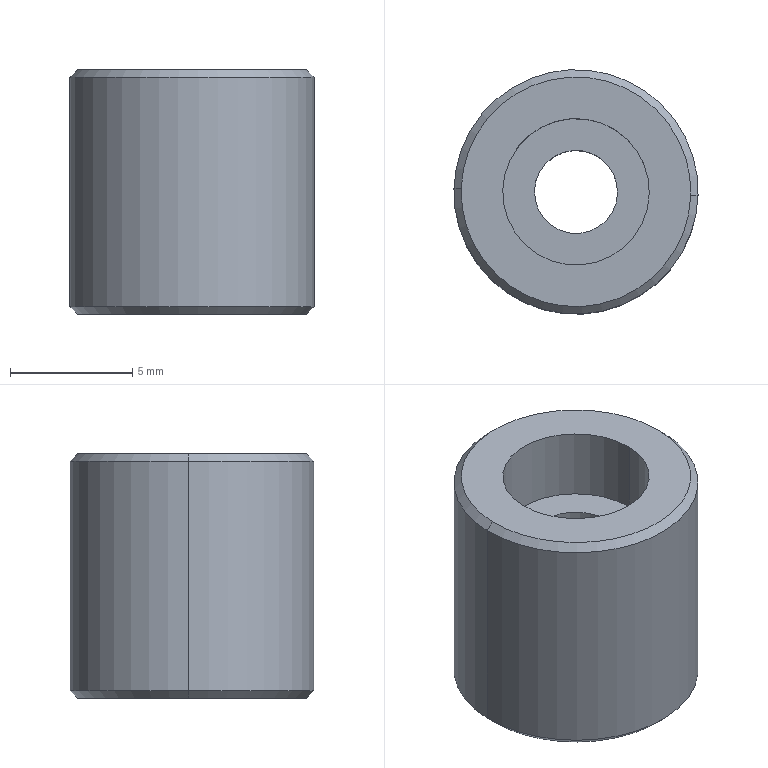Component | SolidWorks | DZ.KX.203-TC1505-20-18-05-90-1 | 1 solid | 15 faces | box 10 x 10 x 10 mm | volume 623 mm3 | cone 6 | cylinder 6 | plane 3 | commonest cylinder face diameters 3.4 x2 6 x2 10 x2 | material Plain Carbon Steel
build123d program:
from build123d import *

# Parameters (mm, degrees)
SKETCH1_R                                            = 5
BOSS_EXTRUDE1_DEPTH                                  = 10
F_6_0_6_DIAMETER_HOLE1_D                             = 6
F_6_0_6_DIAMETER_HOLE1_DEPTH                         = 3
HOLE_SIZE_SLOTTED_RAISED_COUNTERSUNK_SCR_D           = 3.4
HOLE_SIZE_SLOTTED_RAISED_COUNTERSUNK_SCR_CSINK_D     = 6
HOLE_SIZE_SLOTTED_RAISED_COUNTERSUNK_SCR_CSINK_ANGLE = 90
CHAMFER1_SIZE                                        = 0.3


with BuildPart() as part:
    # Sketch1 → Boss-Extrude1 (new body)
    with BuildSketch(Plane(origin=(0, 0, 0), x_dir=(0, 0, -1), z_dir=(1, 0, 0))):
        Circle(SKETCH1_R)
    extrude(amount=BOSS_EXTRUDE1_DEPTH)

    # 6.0 _6_ Diameter Hole1
    with Locations(Plane(origin=(10, 0, 0), x_dir=(0, 0, -1), z_dir=(1, 0, 0))):
        with Locations((0, 0)):
            Hole(F_6_0_6_DIAMETER_HOLE1_D / 2, depth=F_6_0_6_DIAMETER_HOLE1_DEPTH)

    # Hole Size Slotted Raised Countersunk Scr (through all)
    with Locations(Plane.ZY):
        with Locations((0, 0)):
            CounterSinkHole(HOLE_SIZE_SLOTTED_RAISED_COUNTERSUNK_SCR_D / 2, HOLE_SIZE_SLOTTED_RAISED_COUNTERSUNK_SCR_CSINK_D / 2, counter_sink_angle=HOLE_SIZE_SLOTTED_RAISED_COUNTERSUNK_SCR_CSINK_ANGLE)

    # Chamfer1
    chamfer1_edges = [part.edges().sort_by_distance(p)[0] for p in [
        (0, 0, 5),
        (10, 0, 5),
    ]]
    chamfer(chamfer1_edges, length=CHAMFER1_SIZE)


solid = part.part

# Placed as in the assembly
solid = solid.moved(Location((295.5, -817.807, 17.06), (0, -90, 0)))
STEP:
#1=COLOUR_RGB('',0.7922,0.8196,0.9333);
#2=FILL_AREA_STYLE_COLOUR('',#1);
#3=FILL_AREA_STYLE('',(#2));
#4=SURFACE_STYLE_FILL_AREA(#3);
#5=SURFACE_SIDE_STYLE('',(#4));
#6=SURFACE_STYLE_USAGE(.BOTH.,#5);
#7=PRESENTATION_STYLE_ASSIGNMENT((#6));
#8=CARTESIAN_POINT('',(11.819,-32.203,1.065));
#9=VERTEX_POINT('',#8);
#10=CARTESIAN_POINT('',(11.449,-32.192,1.065));
#11=VERTEX_POINT('',#10);
#12=CARTESIAN_POINT('',(11.634,-32.197,1.065));
#13=DIRECTION('',(0.,0.,1.));
#14=DIRECTION('',(0.9996,-0.02934,0.));
#15=AXIS2_PLACEMENT_3D('',#12,#13,#14);
#16=CIRCLE('',#15,0.185);
#17=EDGE_CURVE('',#9,#11,#16,.T.);
#18=ORIENTED_EDGE('',*,*,#17,.F.);
#19=CARTESIAN_POINT('',(11.831,-32.203,1.054));
#20=VERTEX_POINT('',#19);
#21=CARTESIAN_POINT('',(11.819,-32.203,1.065));
#22=DIRECTION('',(0.7068,-0.02075,-0.7071));
#23=VECTOR('',#22,39.37);
#24=LINE('',#21,#23);
#25=EDGE_CURVE('',#9,#20,#24,.T.);
#26=ORIENTED_EDGE('',*,*,#25,.T.);
#27=CARTESIAN_POINT('',(11.437,-32.191,1.054));
#28=VERTEX_POINT('',#27);
#29=CARTESIAN_POINT('',(11.634,-32.197,1.054));
#30=DIRECTION('',(-0.,-0.,-1.));
#31=DIRECTION('',(0.9996,-0.02934,0.));
#32=AXIS2_PLACEMENT_3D('',#29,#30,#31);
#33=CIRCLE('',#32,0.1969);
#34=EDGE_CURVE('',#28,#20,#33,.T.);
#35=ORIENTED_EDGE('',*,*,#34,.F.);
#36=CARTESIAN_POINT('',(11.449,-32.192,1.065));
#37=DIRECTION('',(-0.7068,0.02075,-0.7071));
#38=VECTOR('',#37,39.37);
#39=LINE('',#36,#38);
#40=EDGE_CURVE('',#11,#28,#39,.T.);
#41=ORIENTED_EDGE('',*,*,#40,.F.);
#42=EDGE_LOOP('',(#18,#26,#35,#41));
#43=FACE_OUTER_BOUND('',#42,.T.);
#44=CARTESIAN_POINT('',(11.634,-32.197,1.065));
#45=DIRECTION('',(-0.,-0.,-1.));
#46=DIRECTION('',(-0.9996,0.02934,0.));
#47=AXIS2_PLACEMENT_3D('',#44,#45,#46);
#48=CONICAL_SURFACE('',#47,0.185,0.7854);
#49=ADVANCED_FACE('',(#43),#48,.T.);
#50=CARTESIAN_POINT('',(11.449,-32.192,0.6716));
#51=VERTEX_POINT('',#50);
#52=CARTESIAN_POINT('',(11.819,-32.203,0.6716));
#53=VERTEX_POINT('',#52);
#54=CARTESIAN_POINT('',(11.634,-32.197,0.6716));
#55=DIRECTION('',(-0.,-0.,-1.));
#56=DIRECTION('',(0.9996,-0.02934,0.));
#57=AXIS2_PLACEMENT_3D('',#54,#55,#56);
#58=CIRCLE('',#57,0.185);
#59=EDGE_CURVE('',#51,#53,#58,.T.);
#60=ORIENTED_EDGE('',*,*,#59,.F.);
#61=CARTESIAN_POINT('',(11.437,-32.191,0.6834));
#62=VERTEX_POINT('',#61);
#63=CARTESIAN_POINT('',(11.437,-32.191,0.6834));
#64=DIRECTION('',(-0.7068,0.02075,0.7071));
#65=VECTOR('',#64,39.37);
#66=LINE('',#63,#65);
#67=EDGE_CURVE('',#51,#62,#66,.T.);
#68=ORIENTED_EDGE('',*,*,#67,.T.);
#69=CARTESIAN_POINT('',(11.831,-32.203,0.6834));
#70=VERTEX_POINT('',#69);
#71=CARTESIAN_POINT('',(11.634,-32.197,0.6834));
#72=DIRECTION('',(0.,0.,1.));
#73=DIRECTION('',(0.9996,-0.02934,0.));
#74=AXIS2_PLACEMENT_3D('',#71,#72,#73);
#75=CIRCLE('',#74,0.1969);
#76=EDGE_CURVE('',#70,#62,#75,.T.);
#77=ORIENTED_EDGE('',*,*,#76,.F.);
#78=CARTESIAN_POINT('',(11.831,-32.203,0.6834));
#79=DIRECTION('',(0.7068,-0.02075,0.7071));
#80=VECTOR('',#79,39.37);
#81=LINE('',#78,#80);
#82=EDGE_CURVE('',#53,#70,#81,.T.);
#83=ORIENTED_EDGE('',*,*,#82,.F.);
#84=EDGE_LOOP('',(#60,#68,#77,#83));
#85=FACE_OUTER_BOUND('',#84,.T.);
#86=CARTESIAN_POINT('',(11.634,-32.197,0.6834));
#87=DIRECTION('',(0.,0.,1.));
#88=DIRECTION('',(0.9996,-0.02934,0.));
#89=AXIS2_PLACEMENT_3D('',#86,#87,#88);
#90=CONICAL_SURFACE('',#89,0.1969,0.7854);
#91=ADVANCED_FACE('',(#85),#90,.T.);
#92=CARTESIAN_POINT('',(11.701,-32.199,0.7228));
#93=VERTEX_POINT('',#92);
#94=CARTESIAN_POINT('',(11.567,-32.195,0.7228));
#95=VERTEX_POINT('',#94);
#96=CARTESIAN_POINT('',(11.634,-32.197,0.7228));
#97=DIRECTION('',(-0.,-0.,-1.));
#98=DIRECTION('',(-0.9996,0.02934,0.));
#99=AXIS2_PLACEMENT_3D('',#96,#97,#98);
#100=CIRCLE('',#99,0.06693);
#101=EDGE_CURVE('',#93,#95,#100,.T.);
#102=ORIENTED_EDGE('',*,*,#101,.F.);
#103=CARTESIAN_POINT('',(11.752,-32.201,0.6716));
#104=VERTEX_POINT('',#103);
#105=CARTESIAN_POINT('',(11.752,-32.201,0.6716));
#106=DIRECTION('',(0.7068,-0.02075,-0.7071));
#107=VECTOR('',#106,39.37);
#108=LINE('',#105,#107);
#109=EDGE_CURVE('',#93,#104,#108,.T.);
#110=ORIENTED_EDGE('',*,*,#109,.T.);
#111=CARTESIAN_POINT('',(11.516,-32.194,0.6716));
#112=VERTEX_POINT('',#111);
#113=CARTESIAN_POINT('',(11.634,-32.197,0.6716));
#114=DIRECTION('',(-0.,-0.,-1.));
#115=DIRECTION('',(-0.9996,0.02934,0.));
#116=AXIS2_PLACEMENT_3D('',#113,#114,#115);
#117=CIRCLE('',#116,0.1181);
#118=EDGE_CURVE('',#104,#112,#117,.T.);
#119=ORIENTED_EDGE('',*,*,#118,.T.);
#120=CARTESIAN_POINT('',(11.516,-32.194,0.6716));
#121=DIRECTION('',(-0.7068,0.02075,-0.7071));
#122=VECTOR('',#121,39.37);
#123=LINE('',#120,#122);
#124=EDGE_CURVE('',#95,#112,#123,.T.);
#125=ORIENTED_EDGE('',*,*,#124,.F.);
#126=EDGE_LOOP('',(#102,#110,#119,#125));
#127=FACE_OUTER_BOUND('',#126,.T.);
#128=CARTESIAN_POINT('',(11.634,-32.197,0.6716));
#129=DIRECTION('',(-0.,-0.,-1.));
#130=DIRECTION('',(-0.9996,0.02934,0.));
#131=AXIS2_PLACEMENT_3D('',#128,#129,#130);
#132=CONICAL_SURFACE('',#131,0.1181,0.7854);
#133=ADVANCED_FACE('',(#127),#132,.F.);
#134=CARTESIAN_POINT('',(11.701,-32.199,0.9472));
#135=VERTEX_POINT('',#134);
#136=CARTESIAN_POINT('',(11.567,-32.195,0.9472));
#137=VERTEX_POINT('',#136);
#138=CARTESIAN_POINT('',(11.634,-32.197,0.9472));
#139=DIRECTION('',(-0.,-0.,-1.));
#140=DIRECTION('',(-0.9996,0.02934,0.));
#141=AXIS2_PLACEMENT_3D('',#138,#139,#140);
#142=CIRCLE('',#141,0.06693);
#143=EDGE_CURVE('',#135,#137,#142,.T.);
#144=ORIENTED_EDGE('',*,*,#143,.F.);
#145=CARTESIAN_POINT('',(11.701,-32.199,0.6716));
#146=DIRECTION('',(-0.,-0.,-1.));
#147=VECTOR('',#146,39.37);
#148=LINE('',#145,#147);
#149=EDGE_CURVE('',#135,#93,#148,.T.);
#150=ORIENTED_EDGE('',*,*,#149,.T.);
#151=ORIENTED_EDGE('',*,*,#101,.T.);
#152=CARTESIAN_POINT('',(11.567,-32.195,0.6716));
#153=DIRECTION('',(-0.,-0.,-1.));
#154=VECTOR('',#153,39.37);
#155=LINE('',#152,#154);
#156=EDGE_CURVE('',#137,#95,#155,.T.);
#157=ORIENTED_EDGE('',*,*,#156,.F.);
#158=EDGE_LOOP('',(#144,#150,#151,#157));
#159=FACE_OUTER_BOUND('',#158,.T.);
#160=CARTESIAN_POINT('',(11.634,-32.197,0.6716));
#161=DIRECTION('',(-0.,-0.,-1.));
#162=DIRECTION('',(-0.9996,0.02934,0.));
#163=AXIS2_PLACEMENT_3D('',#160,#161,#162);
#164=CYLINDRICAL_SURFACE('',#163,0.06693);
#165=ADVANCED_FACE('',(#159),#164,.F.);
#166=CARTESIAN_POINT('',(11.516,-32.194,0.9472));
#167=VERTEX_POINT('',#166);
#168=CARTESIAN_POINT('',(11.752,-32.201,0.9472));
#169=VERTEX_POINT('',#168);
#170=CARTESIAN_POINT('',(11.634,-32.197,0.9472));
#171=DIRECTION('',(0.,0.,1.));
#172=DIRECTION('',(0.9996,-0.02934,0.));
#173=AXIS2_PLACEMENT_3D('',#170,#171,#172);
#174=CIRCLE('',#173,0.1181);
#175=EDGE_CURVE('',#167,#169,#174,.T.);
#176=ORIENTED_EDGE('',*,*,#175,.F.);
#177=CARTESIAN_POINT('',(11.516,-32.194,1.065));
#178=VERTEX_POINT('',#177);
#179=CARTESIAN_POINT('',(11.516,-32.194,1.065));
#180=DIRECTION('',(0.,0.,1.));
#181=VECTOR('',#180,39.37);
#182=LINE('',#179,#181);
#183=EDGE_CURVE('',#167,#178,#182,.T.);
#184=ORIENTED_EDGE('',*,*,#183,.T.);
#185=CARTESIAN_POINT('',(11.752,-32.201,1.065));
#186=VERTEX_POINT('',#185);
#187=CARTESIAN_POINT('',(11.634,-32.197,1.065));
#188=DIRECTION('',(0.,0.,1.));
#189=DIRECTION('',(0.9996,-0.02934,0.));
#190=AXIS2_PLACEMENT_3D('',#187,#188,#189);
#191=CIRCLE('',#190,0.1181);
#192=EDGE_CURVE('',#178,#186,#191,.T.);
#193=ORIENTED_EDGE('',*,*,#192,.T.);
#194=CARTESIAN_POINT('',(11.752,-32.201,1.065));
#195=DIRECTION('',(0.,0.,1.));
#196=VECTOR('',#195,39.37);
#197=LINE('',#194,#196);
#198=EDGE_CURVE('',#169,#186,#197,.T.);
#199=ORIENTED_EDGE('',*,*,#198,.F.);
#200=EDGE_LOOP('',(#176,#184,#193,#199));
#201=FACE_OUTER_BOUND('',#200,.T.);
#202=CARTESIAN_POINT('',(11.634,-32.197,1.065));
#203=DIRECTION('',(0.,0.,1.));
#204=DIRECTION('',(0.9996,-0.02934,0.));
#205=AXIS2_PLACEMENT_3D('',#202,#203,#204);
#206=CYLINDRICAL_SURFACE('',#205,0.1181);
#207=ADVANCED_FACE('',(#201),#206,.F.);
#208=ORIENTED_EDGE('',*,*,#34,.T.);
#209=CARTESIAN_POINT('',(11.831,-32.203,1.065));
#210=DIRECTION('',(-0.,-0.,-1.));
#211=VECTOR('',#210,39.37);
#212=LINE('',#209,#211);
#213=EDGE_CURVE('',#20,#70,#212,.T.);
#214=ORIENTED_EDGE('',*,*,#213,.T.);
#215=ORIENTED_EDGE('',*,*,#76,.T.);
#216=CARTESIAN_POINT('',(11.437,-32.191,1.065));
#217=DIRECTION('',(-0.,-0.,-1.));
#218=VECTOR('',#217,39.37);
#219=LINE('',#216,#218);
#220=EDGE_CURVE('',#28,#62,#219,.T.);
#221=ORIENTED_EDGE('',*,*,#220,.F.);
#222=EDGE_LOOP('',(#208,#214,#215,#221));
#223=FACE_OUTER_BOUND('',#222,.T.);
#224=CARTESIAN_POINT('',(11.634,-32.197,1.065));
#225=DIRECTION('',(-0.,-0.,-1.));
#226=DIRECTION('',(-0.9996,0.02934,0.));
#227=AXIS2_PLACEMENT_3D('',#224,#225,#226);
#228=CYLINDRICAL_SURFACE('',#227,0.1969);
#229=ADVANCED_FACE('',(#223),#228,.T.);
#230=ORIENTED_EDGE('',*,*,#213,.F.);
#231=CARTESIAN_POINT('',(11.634,-32.197,1.054));
#232=DIRECTION('',(-0.,-0.,-1.));
#233=DIRECTION('',(0.9996,-0.02934,0.));
#234=AXIS2_PLACEMENT_3D('',#231,#232,#233);
#235=CIRCLE('',#234,0.1969);
#236=EDGE_CURVE('',#20,#28,#235,.T.);
#237=ORIENTED_EDGE('',*,*,#236,.T.);
#238=ORIENTED_EDGE('',*,*,#220,.T.);
#239=CARTESIAN_POINT('',(11.634,-32.197,0.6834));
#240=DIRECTION('',(0.,0.,1.));
#241=DIRECTION('',(0.9996,-0.02934,0.));
#242=AXIS2_PLACEMENT_3D('',#239,#240,#241);
#243=CIRCLE('',#242,0.1969);
#244=EDGE_CURVE('',#62,#70,#243,.T.);
#245=ORIENTED_EDGE('',*,*,#244,.T.);
#246=EDGE_LOOP('',(#230,#237,#238,#245));
#247=FACE_OUTER_BOUND('',#246,.T.);
#248=CARTESIAN_POINT('',(11.634,-32.197,1.065));
#249=DIRECTION('',(-0.,-0.,-1.));
#250=DIRECTION('',(-0.9996,0.02934,0.));
#251=AXIS2_PLACEMENT_3D('',#248,#249,#250);
#252=CYLINDRICAL_SURFACE('',#251,0.1969);
#253=ADVANCED_FACE('',(#247),#252,.T.);
#254=CARTESIAN_POINT('',(11.634,-32.197,1.065));
#255=DIRECTION('',(0.,0.,1.));
#256=DIRECTION('',(0.9996,-0.02934,0.));
#257=AXIS2_PLACEMENT_3D('',#254,#255,#256);
#258=CIRCLE('',#257,0.185);
#259=EDGE_CURVE('',#11,#9,#258,.T.);
#260=ORIENTED_EDGE('',*,*,#259,.T.);
#261=ORIENTED_EDGE('',*,*,#17,.T.);
#262=EDGE_LOOP('',(#260,#261));
#263=FACE_OUTER_BOUND('',#262,.T.);
#264=CARTESIAN_POINT('',(11.634,-32.197,1.065));
#265=DIRECTION('',(0.,0.,1.));
#266=DIRECTION('',(0.9996,-0.02934,0.));
#267=AXIS2_PLACEMENT_3D('',#264,#265,#266);
#268=CIRCLE('',#267,0.1181);
#269=EDGE_CURVE('',#186,#178,#268,.T.);
#270=ORIENTED_EDGE('',*,*,#269,.F.);
#271=ORIENTED_EDGE('',*,*,#192,.F.);
#272=EDGE_LOOP('',(#270,#271));
#273=FACE_BOUND('',#272,.T.);
#274=CARTESIAN_POINT('',(11.634,-32.197,1.065));
#275=DIRECTION('',(0.,0.,1.));
#276=DIRECTION('',(0.9996,-0.02934,0.));
#277=AXIS2_PLACEMENT_3D('',#274,#275,#276);
#278=PLANE('',#277);
#279=ADVANCED_FACE('',(#263,#273),#278,.T.);
#280=CARTESIAN_POINT('',(11.634,-32.197,0.6716));
#281=DIRECTION('',(-0.,-0.,-1.));
#282=DIRECTION('',(0.9996,-0.02934,0.));
#283=AXIS2_PLACEMENT_3D('',#280,#281,#282);
#284=CIRCLE('',#283,0.185);
#285=EDGE_CURVE('',#53,#51,#284,.T.);
#286=ORIENTED_EDGE('',*,*,#285,.T.);
#287=ORIENTED_EDGE('',*,*,#59,.T.);
#288=EDGE_LOOP('',(#286,#287));
#289=FACE_OUTER_BOUND('',#288,.T.);
#290=CARTESIAN_POINT('',(11.634,-32.197,0.6716));
#291=DIRECTION('',(-0.,-0.,-1.));
#292=DIRECTION('',(-0.9996,0.02934,0.));
#293=AXIS2_PLACEMENT_3D('',#290,#291,#292);
#294=CIRCLE('',#293,0.1181);
#295=EDGE_CURVE('',#112,#104,#294,.T.);
#296=ORIENTED_EDGE('',*,*,#295,.F.);
#297=ORIENTED_EDGE('',*,*,#118,.F.);
#298=EDGE_LOOP('',(#296,#297));
#299=FACE_BOUND('',#298,.T.);
#300=CARTESIAN_POINT('',(11.634,-32.197,0.6716));
#301=DIRECTION('',(0.,0.,1.));
#302=DIRECTION('',(0.9996,-0.02934,0.));
#303=AXIS2_PLACEMENT_3D('',#300,#301,#302);
#304=PLANE('',#303);
#305=ADVANCED_FACE('',(#289,#299),#304,.F.);
#306=CARTESIAN_POINT('',(11.634,-32.197,0.9472));
#307=DIRECTION('',(-0.,-0.,-1.));
#308=DIRECTION('',(-0.9996,0.02934,0.));
#309=AXIS2_PLACEMENT_3D('',#306,#307,#308);
#310=CIRCLE('',#309,0.06693);
#311=EDGE_CURVE('',#137,#135,#310,.T.);
#312=ORIENTED_EDGE('',*,*,#311,.T.);
#313=ORIENTED_EDGE('',*,*,#143,.T.);
#314=EDGE_LOOP('',(#312,#313));
#315=FACE_BOUND('',#314,.T.);
#316=CARTESIAN_POINT('',(11.634,-32.197,0.9472));
#317=DIRECTION('',(0.,0.,1.));
#318=DIRECTION('',(0.9996,-0.02934,0.));
#319=AXIS2_PLACEMENT_3D('',#316,#317,#318);
#320=CIRCLE('',#319,0.1181);
#321=EDGE_CURVE('',#169,#167,#320,.T.);
#322=ORIENTED_EDGE('',*,*,#321,.T.);
#323=ORIENTED_EDGE('',*,*,#175,.T.);
#324=EDGE_LOOP('',(#322,#323));
#325=FACE_OUTER_BOUND('',#324,.T.);
#326=CARTESIAN_POINT('',(11.634,-32.197,0.9472));
#327=DIRECTION('',(-0.,-0.,-1.));
#328=DIRECTION('',(-0.9996,0.02934,-0.));
#329=AXIS2_PLACEMENT_3D('',#326,#327,#328);
#330=PLANE('',#329);
#331=ADVANCED_FACE('',(#315,#325),#330,.F.);
#332=ORIENTED_EDGE('',*,*,#183,.F.);
#333=ORIENTED_EDGE('',*,*,#321,.F.);
#334=ORIENTED_EDGE('',*,*,#198,.T.);
#335=ORIENTED_EDGE('',*,*,#269,.T.);
#336=EDGE_LOOP('',(#332,#333,#334,#335));
#337=FACE_OUTER_BOUND('',#336,.T.);
#338=CARTESIAN_POINT('',(11.634,-32.197,1.065));
#339=DIRECTION('',(0.,0.,1.));
#340=DIRECTION('',(0.9996,-0.02934,0.));
#341=AXIS2_PLACEMENT_3D('',#338,#339,#340);
#342=CYLINDRICAL_SURFACE('',#341,0.1181);
#343=ADVANCED_FACE('',(#337),#342,.F.);
#344=ORIENTED_EDGE('',*,*,#149,.F.);
#345=ORIENTED_EDGE('',*,*,#311,.F.);
#346=ORIENTED_EDGE('',*,*,#156,.T.);
#347=CARTESIAN_POINT('',(11.634,-32.197,0.7228));
#348=DIRECTION('',(-0.,-0.,-1.));
#349=DIRECTION('',(-0.9996,0.02934,0.));
#350=AXIS2_PLACEMENT_3D('',#347,#348,#349);
#351=CIRCLE('',#350,0.06693);
#352=EDGE_CURVE('',#95,#93,#351,.T.);
#353=ORIENTED_EDGE('',*,*,#352,.T.);
#354=EDGE_LOOP('',(#344,#345,#346,#353));
#355=FACE_OUTER_BOUND('',#354,.T.);
#356=CARTESIAN_POINT('',(11.634,-32.197,0.6716));
#357=DIRECTION('',(-0.,-0.,-1.));
#358=DIRECTION('',(-0.9996,0.02934,0.));
#359=AXIS2_PLACEMENT_3D('',#356,#357,#358);
#360=CYLINDRICAL_SURFACE('',#359,0.06693);
#361=ADVANCED_FACE('',(#355),#360,.F.);
#362=ORIENTED_EDGE('',*,*,#109,.F.);
#363=ORIENTED_EDGE('',*,*,#352,.F.);
#364=ORIENTED_EDGE('',*,*,#124,.T.);
#365=ORIENTED_EDGE('',*,*,#295,.T.);
#366=EDGE_LOOP('',(#362,#363,#364,#365));
#367=FACE_OUTER_BOUND('',#366,.T.);
#368=CARTESIAN_POINT('',(11.634,-32.197,0.6716));
#369=DIRECTION('',(-0.,-0.,-1.));
#370=DIRECTION('',(-0.9996,0.02934,0.));
#371=AXIS2_PLACEMENT_3D('',#368,#369,#370);
#372=CONICAL_SURFACE('',#371,0.1181,0.7854);
#373=ADVANCED_FACE('',(#367),#372,.F.);
#374=ORIENTED_EDGE('',*,*,#67,.F.);
#375=ORIENTED_EDGE('',*,*,#285,.F.);
#376=ORIENTED_EDGE('',*,*,#82,.T.);
#377=ORIENTED_EDGE('',*,*,#244,.F.);
#378=EDGE_LOOP('',(#374,#375,#376,#377));
#379=FACE_OUTER_BOUND('',#378,.T.);
#380=CARTESIAN_POINT('',(11.634,-32.197,0.6834));
#381=DIRECTION('',(0.,0.,1.));
#382=DIRECTION('',(0.9996,-0.02934,0.));
#383=AXIS2_PLACEMENT_3D('',#380,#381,#382);
#384=CONICAL_SURFACE('',#383,0.1969,0.7854);
#385=ADVANCED_FACE('',(#379),#384,.T.);
#386=ORIENTED_EDGE('',*,*,#25,.F.);
#387=ORIENTED_EDGE('',*,*,#259,.F.);
#388=ORIENTED_EDGE('',*,*,#40,.T.);
#389=ORIENTED_EDGE('',*,*,#236,.F.);
#390=EDGE_LOOP('',(#386,#387,#388,#389));
#391=FACE_OUTER_BOUND('',#390,.T.);
#392=CARTESIAN_POINT('',(11.634,-32.197,1.065));
#393=DIRECTION('',(-0.,-0.,-1.));
#394=DIRECTION('',(-0.9996,0.02934,0.));
#395=AXIS2_PLACEMENT_3D('',#392,#393,#394);
#396=CONICAL_SURFACE('',#395,0.185,0.7854);
#397=ADVANCED_FACE('',(#391),#396,.T.);
#398=CLOSED_SHELL('',(#49,#91,#133,#165,#207,#229,#253,#279,#305,#331,#343,#361,#373,#385,#397));
#399=MANIFOLD_SOLID_BREP('',#398);
#400=STYLED_ITEM('',(#7),#399);
#401=PRESENTATION_LAYER_ASSIGNMENT('','',(#400));
#402=(LENGTH_UNIT()NAMED_UNIT(*)SI_UNIT($,.METRE.));
#403=LENGTH_MEASURE_WITH_UNIT(LENGTH_MEASURE(0.0254),#402);
#404=DIMENSIONAL_EXPONENTS(1.,0.,0.,0.,0.,0.,0.);
#405=(CONVERSION_BASED_UNIT('',#403)LENGTH_UNIT()NAMED_UNIT(#404));
#406=UNCERTAINTY_MEASURE_WITH_UNIT(LENGTH_MEASURE(0.00001),#405,'','');
#407=(NAMED_UNIT(*)PLANE_ANGLE_UNIT()SI_UNIT($,.RADIAN.));
#408=(NAMED_UNIT(*)SI_UNIT($,.STERADIAN.)SOLID_ANGLE_UNIT());
#409=(GEOMETRIC_REPRESENTATION_CONTEXT(3)GLOBAL_UNCERTAINTY_ASSIGNED_CONTEXT((#406))GLOBAL_UNIT_ASSIGNED_CONTEXT((#405,#407,#408))REPRESENTATION_CONTEXT('',''));
#410=MECHANICAL_DESIGN_GEOMETRIC_PRESENTATION_REPRESENTATION('',(#400),#409);
#411=CARTESIAN_POINT('',(0.,0.,0.));
#412=DIRECTION('',(0.,0.,1.));
#413=DIRECTION('',(1.,0.,0.));
#414=AXIS2_PLACEMENT_3D('',#411,#412,#413);
#415=(LENGTH_UNIT()NAMED_UNIT(*)SI_UNIT($,.METRE.));
#416=LENGTH_MEASURE_WITH_UNIT(LENGTH_MEASURE(0.0254),#415);
#417=DIMENSIONAL_EXPONENTS(1.,0.,0.,0.,0.,0.,0.);
#418=(CONVERSION_BASED_UNIT('',#416)LENGTH_UNIT()NAMED_UNIT(#417));
#419=UNCERTAINTY_MEASURE_WITH_UNIT(LENGTH_MEASURE(0.00001),#418,'','');
#420=(NAMED_UNIT(*)PLANE_ANGLE_UNIT()SI_UNIT($,.RADIAN.));
#421=(NAMED_UNIT(*)SI_UNIT($,.STERADIAN.)SOLID_ANGLE_UNIT());
#422=(GEOMETRIC_REPRESENTATION_CONTEXT(3)GLOBAL_UNCERTAINTY_ASSIGNED_CONTEXT((#419))GLOBAL_UNIT_ASSIGNED_CONTEXT((#418,#420,#421))REPRESENTATION_CONTEXT('',''));
#423=ADVANCED_BREP_SHAPE_REPRESENTATION('',(#399,#414),#422);